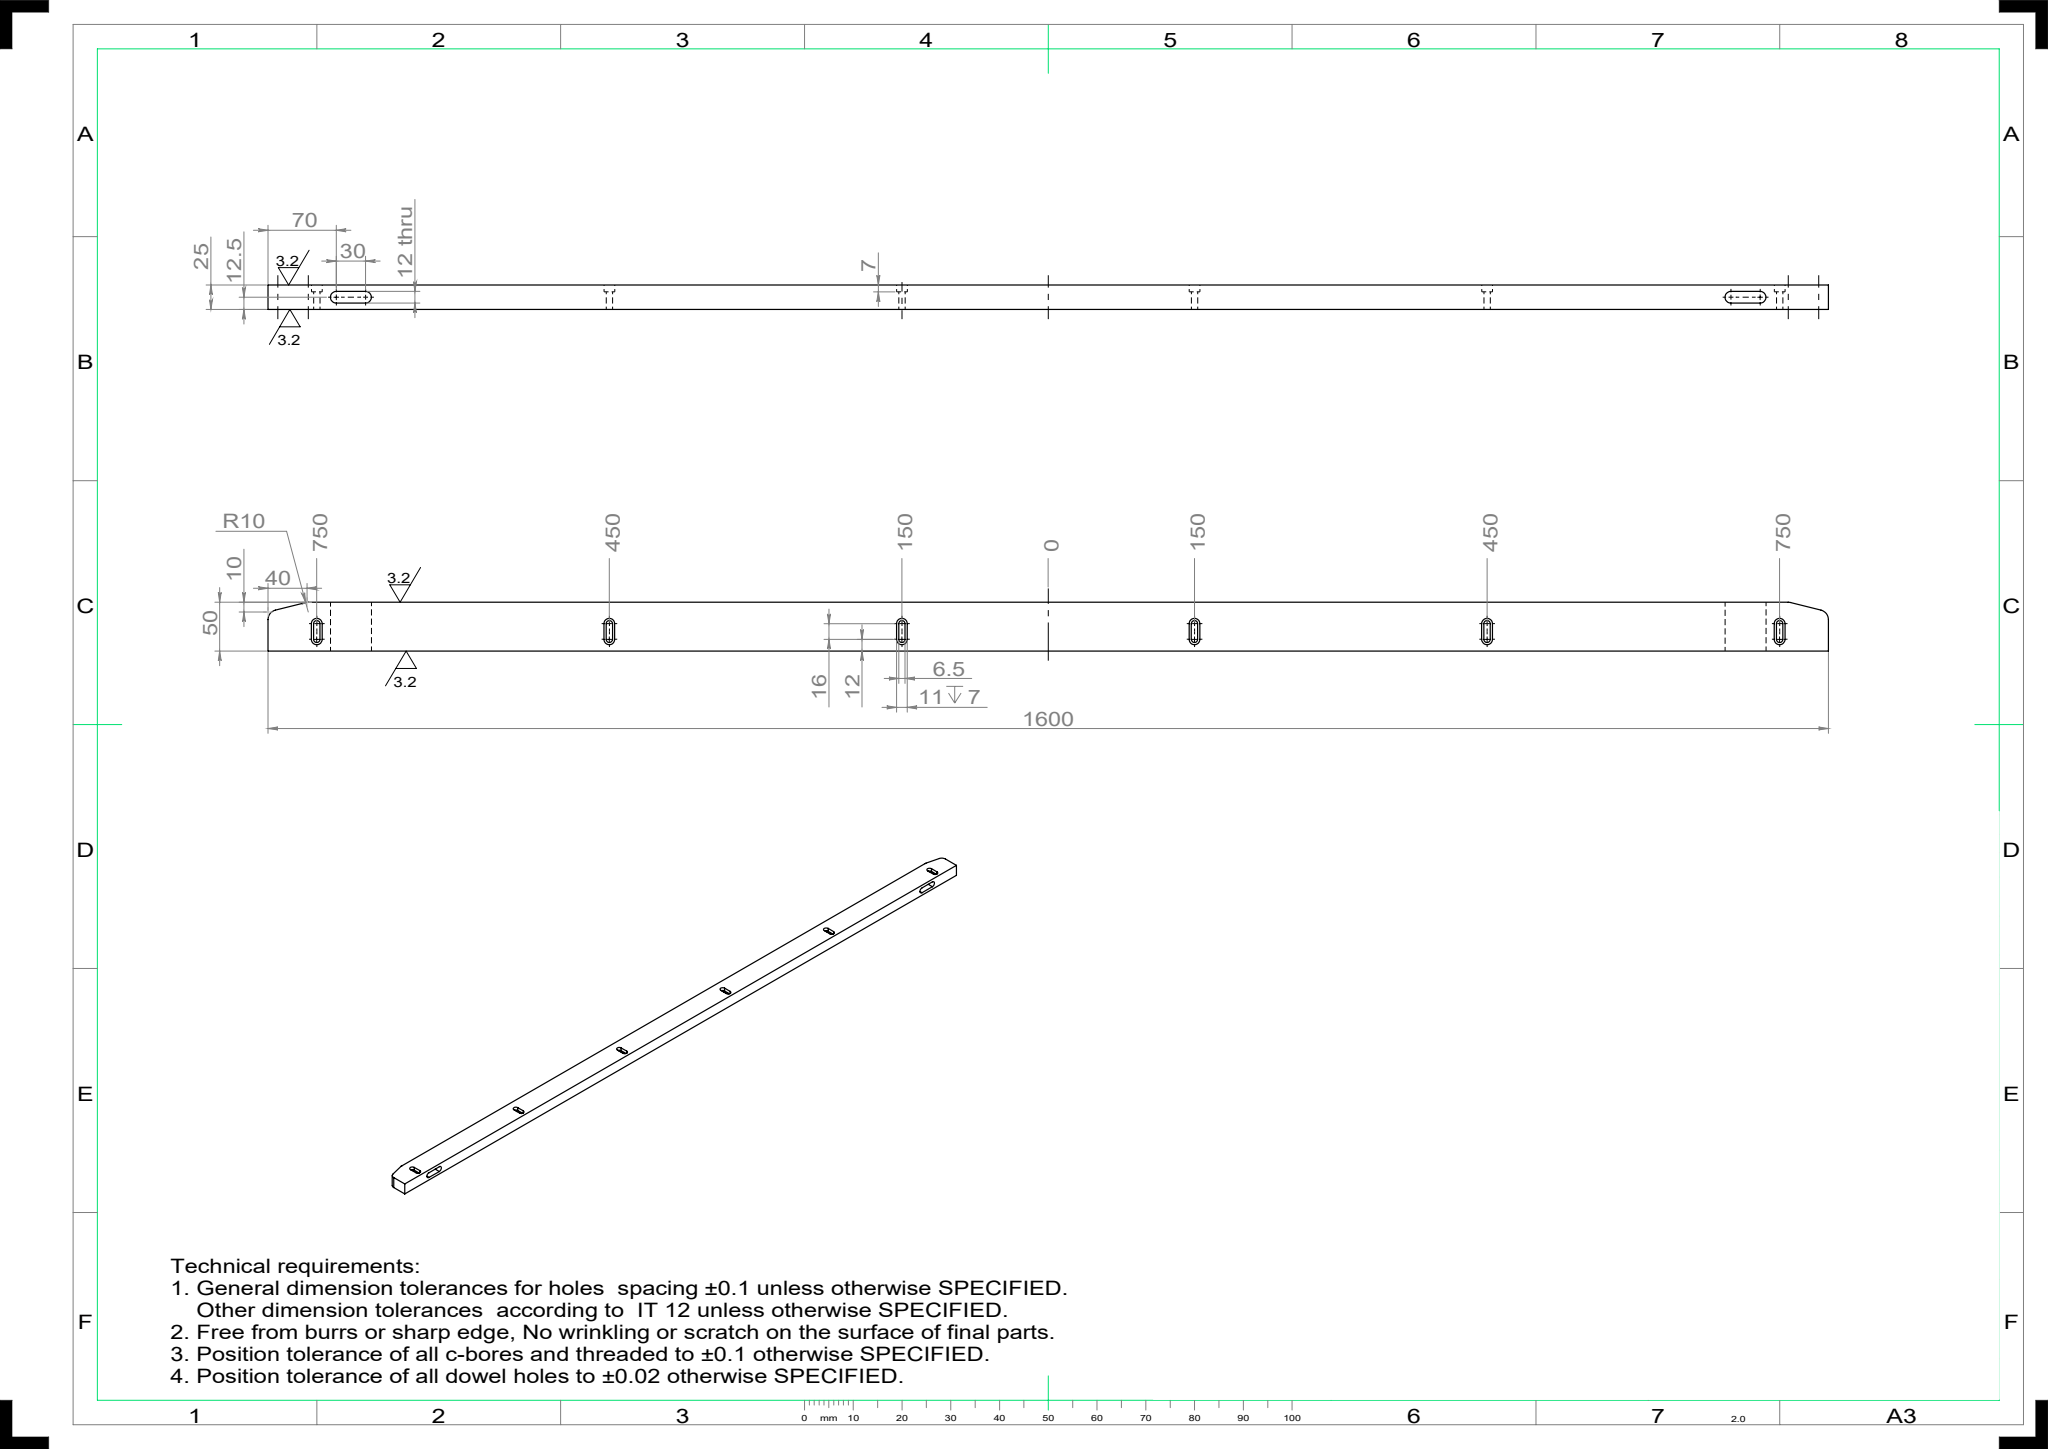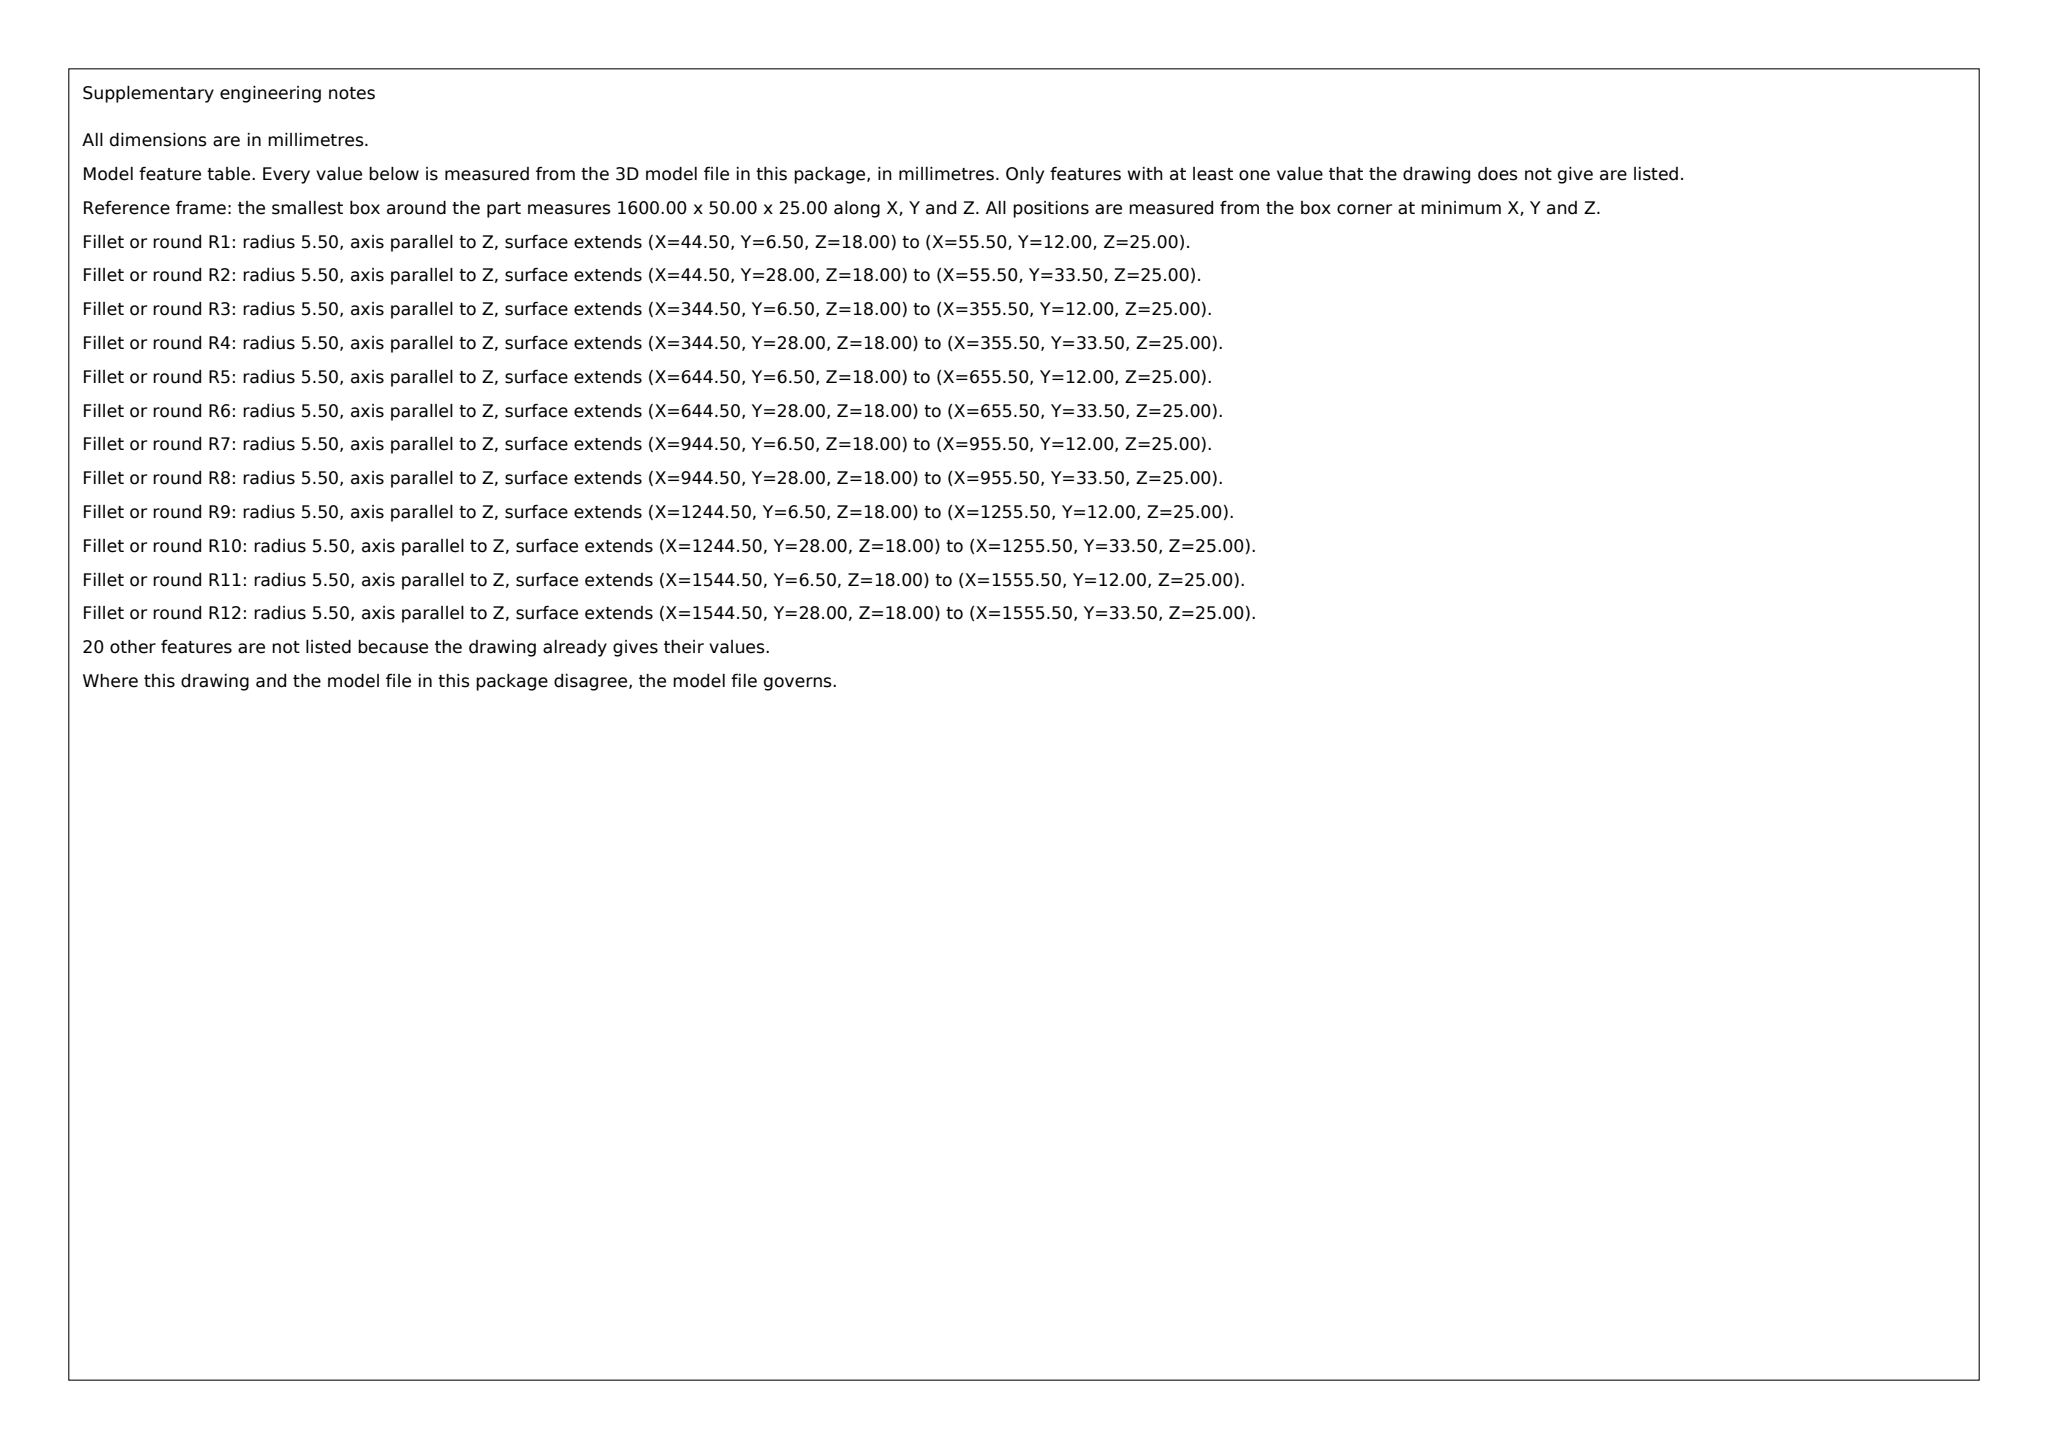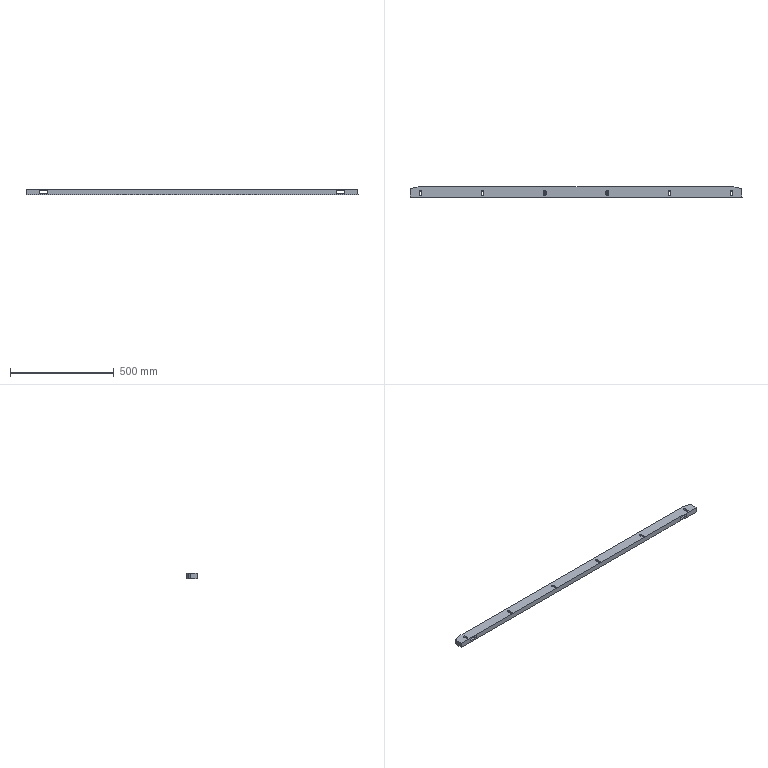Part | SolidWorks | mm | 1 solid | 74 faces | box 1600 x 50 x 25 mm | volume 1915899 mm3 | plane 42 | cylinder 32 | commonest cylinder face diameters 6.5 x12 11 x12 20 x4 12 x4
Drawing notes:
RH END Ø12 THRU SLOT: 70 FROM RH END, 30 C-C (MIRRORS LH END) | from the solid: 12 dia y-axis cylinders at x=1500 & 1530, z=12.5; bbox x=1600 -> 70 & 100 from RH end, 30 apart
RH END CORNER CUT 10 x 40, R10 TANGENT BLENDS (MIRRORS LH END) | from the solid: R10 (dia 20) fillet axes at (1558.77,40) & (1590,32.19); bbox 1600 x 50 -> 40 long x 10 high cut at RH end